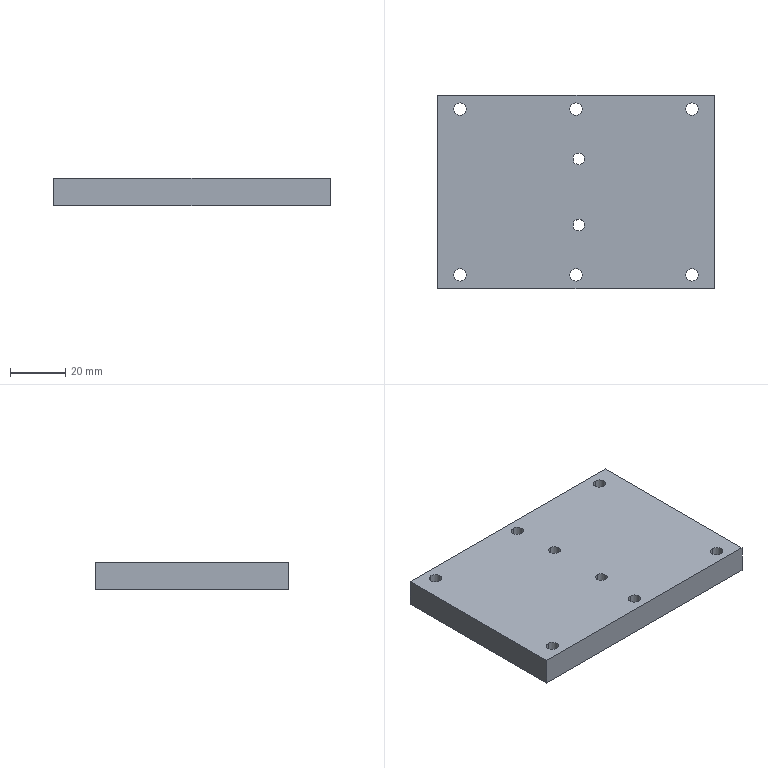Component | SolidWorks | 08-1111-1 | 1 solid | 40 faces | box 100 x 70 x 10 mm | volume 67862 mm3 | cylinder 28 | plane 12 | commonest cylinder face diameters 8 x12 4.5 x12 4.2 x4 | material AL6061
build123d program:
from build123d import *

# Parameters (mm, degrees)
SKETCH1_W                                       = 100
SKETCH1_H                                       = 10
EXTRUDE1_DEPTH                                  = 70
M4_HEX_SOCKET_HEAD_CAP_SCREW_CBORE1_D           = 4.5
M4_HEX_SOCKET_HEAD_CAP_SCREW_CBORE1_CBORE_D     = 8
M4_HEX_SOCKET_HEAD_CAP_SCREW_CBORE1_CBORE_DEPTH = 4.4
M4_HEX_SOCKET_HEAD_CAP_SCREW_CBORE2_D           = 4.5
M4_HEX_SOCKET_HEAD_CAP_SCREW_CBORE2_CBORE_D     = 8
M4_HEX_SOCKET_HEAD_CAP_SCREW_CBORE2_CBORE_DEPTH = 4.4
M5_TAPPED_HOLE1_D                               = 4.2


with BuildPart() as part:
    # Sketch1 → Extrude1 (new body)
    with BuildSketch(Plane.XY):
        with Locations((50, 5)):
            Rectangle(SKETCH1_W, SKETCH1_H)
    extrude(amount=EXTRUDE1_DEPTH)

    # M4 Hex Socket Head Cap Screw CBORE1 (through all)
    with Locations(Plane(origin=(0, 10, 0), x_dir=(-1, 0, 0), z_dir=(0, 1, 0))):
        with Locations((-8, 65), (-50, 65), (-92, 65)):
            CounterBoreHole(M4_HEX_SOCKET_HEAD_CAP_SCREW_CBORE1_D / 2, M4_HEX_SOCKET_HEAD_CAP_SCREW_CBORE1_CBORE_D / 2, M4_HEX_SOCKET_HEAD_CAP_SCREW_CBORE1_CBORE_DEPTH)

    # M4 Hex Socket Head Cap Screw CBORE2 (through all)
    with Locations(Plane(origin=(0, 10, 0), x_dir=(-1, 0, 0), z_dir=(0, 1, 0))):
        with Locations((-8, 5), (-50, 5), (-92, 5)):
            CounterBoreHole(M4_HEX_SOCKET_HEAD_CAP_SCREW_CBORE2_D / 2, M4_HEX_SOCKET_HEAD_CAP_SCREW_CBORE2_CBORE_D / 2, M4_HEX_SOCKET_HEAD_CAP_SCREW_CBORE2_CBORE_DEPTH)

    # M5 Tapped Hole1 (through all)
    with Locations(Plane(origin=(0, 0, 0), x_dir=(-1, 0, 0), z_dir=(0, -1, 0))):
        with Locations((-51, -23), (-51, -47)):
            Hole(M5_TAPPED_HOLE1_D / 2)


solid = part.part

# Placed as in the assembly
solid = solid.moved(Location((-64.57, -10, -66), (-90, 0, 0)))